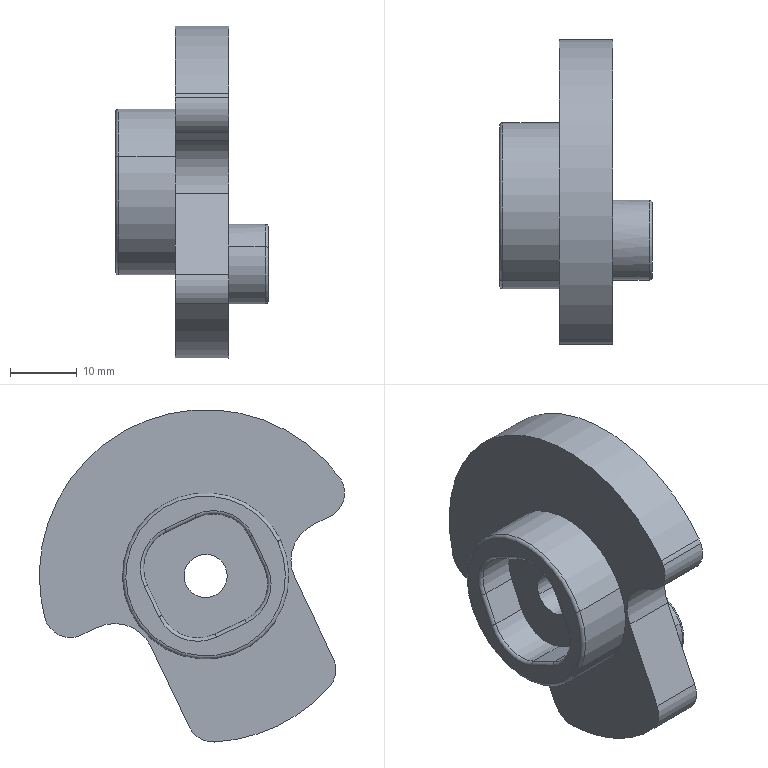Component | SolidWorks | Crank-1 | 1 solid | 55 faces | volume 14987 mm3 | cylinder 27 | plane 14 | torus 12 | cone 2 | commonest cylinder face diameters 12 x8 8 x5 1 x4 5 x2 6.5 x2 11 x2 25 x2 50 x2